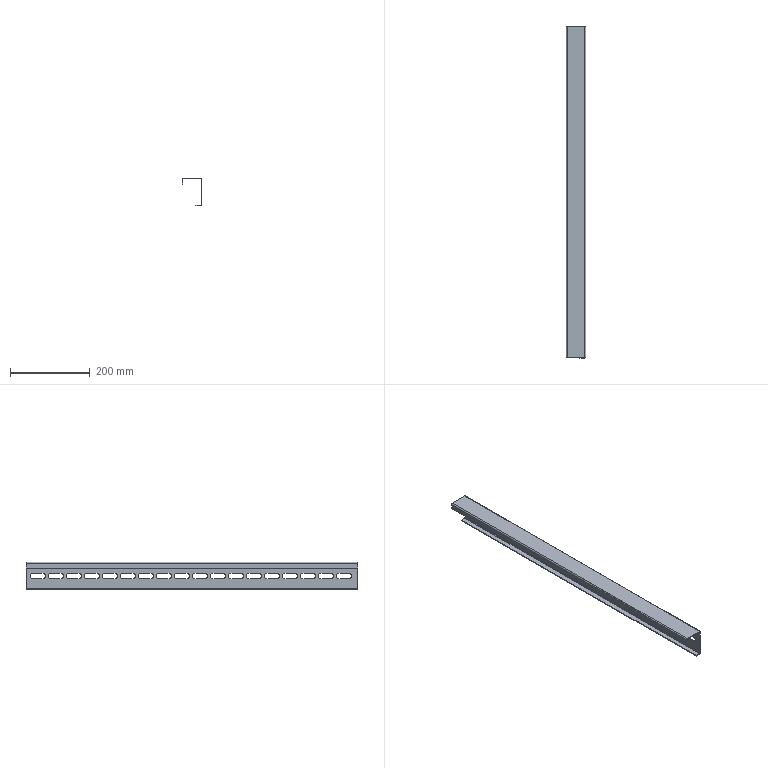Component | SolidWorks | HighVoltageMountingPlateAssembly-2_HighVoltageOutletCabinetMountingPlate-1 | 1 solid | 120 faces | volume 217959 mm3 | cylinder 60 | plane 60 | commonest cylinder face diameters 13.2 x54 6 x3 2 x3 | material Plain Carbon Steel